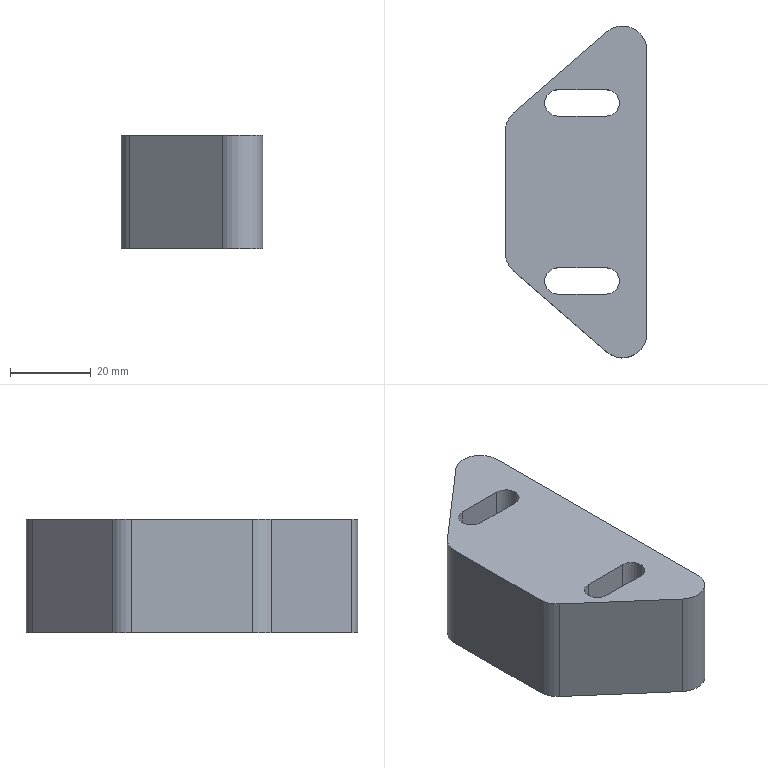Component | SolidWorks | DoubleFilmTransport-1_SynchronousBeltPressureBlock-1 | 1 solid | 19 faces | box 35 x 82 x 28 mm | volume 56182 mm3 | plane 10 | cylinder 9 | commonest cylinder face diameters 12 x5 6.5 x4
build123d program:
from build123d import *

# Parameters (mm, degrees)
BOSS_EXTRUDE1_DEPTH = 28


with BuildPart() as part:
    # Sketch1 → Boss-Extrude1 (new body)
    with BuildSketch(Plane(origin=(0, 0, -14), x_dir=(-1, 0, 0), z_dir=(0, 0, -1))):
        with BuildLine():
            Line((35, 0), (-35, 0))
            ThreePointArc((-35, 0), (-40.46, -3.512), (-39.528, -9.937))
            Line((-39.528, -9.937), (-19.528, -32.937))
            ThreePointArc((-19.528, -32.937), (-17.488, -34.46), (-15, -35))
            Line((-15, -35), (15, -35))
            ThreePointArc((15, -35), (17.488, -34.46), (19.528, -32.937))
            Line((19.528, -32.937), (39.528, -9.937))
            ThreePointArc((39.528, -9.937), (40.46, -3.512), (35, 0))
        make_face()
        with BuildLine():
            Line((18.75, -22), (18.75, -10))
            ThreePointArc((18.75, -10), (22, -6.75), (25.25, -10))
            Line((25.25, -10), (25.25, -22))
            ThreePointArc((25.25, -22), (22, -25.25), (18.75, -22))
        make_face(mode=Mode.SUBTRACT)
        with BuildLine():
            Line((-25.25, -22), (-25.25, -10))
            ThreePointArc((-25.25, -10), (-22, -6.75), (-18.75, -10))
            Line((-18.75, -10), (-18.75, -22))
            ThreePointArc((-18.75, -22), (-22, -25.25), (-25.25, -22))
        make_face(mode=Mode.SUBTRACT)
    extrude(amount=-BOSS_EXTRUDE1_DEPTH)


solid = part.part

# Placed as in the assembly
solid = solid.moved(Location((-356.177, 174.373, 110), (0, 0, -90)))
STEP:
#1=COLOUR_RGB('',0.7922,0.8196,0.9333);
#2=FILL_AREA_STYLE_COLOUR('',#1);
#3=FILL_AREA_STYLE('',(#2));
#4=SURFACE_STYLE_FILL_AREA(#3);
#5=SURFACE_SIDE_STYLE('',(#4));
#6=SURFACE_STYLE_USAGE(.BOTH.,#5);
#7=PRESENTATION_STYLE_ASSIGNMENT((#6));
#8=CARTESIAN_POINT('',(-14.414,8.421,4.882));
#9=VERTEX_POINT('',#8);
#10=CARTESIAN_POINT('',(-14.259,8.479,4.882));
#11=VERTEX_POINT('',#10);
#12=CARTESIAN_POINT('',(-14.259,8.243,4.882));
#13=DIRECTION('',(0.,0.,-1.));
#14=DIRECTION('',(0.,1.,0.));
#15=AXIS2_PLACEMENT_3D('',#12,#13,#14);
#16=CIRCLE('',#15,0.2362);
#17=EDGE_CURVE('',#9,#11,#16,.T.);
#18=ORIENTED_EDGE('',*,*,#17,.T.);
#19=CARTESIAN_POINT('',(-14.259,8.479,3.78));
#20=VERTEX_POINT('',#19);
#21=CARTESIAN_POINT('',(-14.259,8.479,4.882));
#22=DIRECTION('',(0.,0.,-1.));
#23=VECTOR('',#22,39.37);
#24=LINE('',#21,#23);
#25=EDGE_CURVE('',#11,#20,#24,.T.);
#26=ORIENTED_EDGE('',*,*,#25,.T.);
#27=CARTESIAN_POINT('',(-14.414,8.421,3.78));
#28=VERTEX_POINT('',#27);
#29=CARTESIAN_POINT('',(-14.259,8.243,3.78));
#30=DIRECTION('',(0.,0.,-1.));
#31=DIRECTION('',(0.,1.,0.));
#32=AXIS2_PLACEMENT_3D('',#29,#30,#31);
#33=CIRCLE('',#32,0.2362);
#34=EDGE_CURVE('',#28,#20,#33,.T.);
#35=ORIENTED_EDGE('',*,*,#34,.F.);
#36=CARTESIAN_POINT('',(-14.414,8.421,4.882));
#37=DIRECTION('',(0.,0.,-1.));
#38=VECTOR('',#37,39.37);
#39=LINE('',#36,#38);
#40=EDGE_CURVE('',#9,#28,#39,.T.);
#41=ORIENTED_EDGE('',*,*,#40,.F.);
#42=EDGE_LOOP('',(#18,#26,#35,#41));
#43=FACE_OUTER_BOUND('',#42,.T.);
#44=CARTESIAN_POINT('',(-14.259,8.243,4.882));
#45=DIRECTION('',(0.,0.,-1.));
#46=DIRECTION('',(0.,1.,0.));
#47=AXIS2_PLACEMENT_3D('',#44,#45,#46);
#48=CYLINDRICAL_SURFACE('',#47,0.2362);
#49=ADVANCED_FACE('',(#43),#48,.T.);
#50=ORIENTED_EDGE('',*,*,#25,.F.);
#51=CARTESIAN_POINT('',(-14.023,8.243,4.882));
#52=VERTEX_POINT('',#51);
#53=CARTESIAN_POINT('',(-14.259,8.243,4.882));
#54=DIRECTION('',(0.,0.,-1.));
#55=DIRECTION('',(0.,1.,0.));
#56=AXIS2_PLACEMENT_3D('',#53,#54,#55);
#57=CIRCLE('',#56,0.2362);
#58=EDGE_CURVE('',#11,#52,#57,.T.);
#59=ORIENTED_EDGE('',*,*,#58,.T.);
#60=CARTESIAN_POINT('',(-14.023,8.243,3.78));
#61=VERTEX_POINT('',#60);
#62=CARTESIAN_POINT('',(-14.023,8.243,4.882));
#63=DIRECTION('',(0.,0.,-1.));
#64=VECTOR('',#63,39.37);
#65=LINE('',#62,#64);
#66=EDGE_CURVE('',#52,#61,#65,.T.);
#67=ORIENTED_EDGE('',*,*,#66,.T.);
#68=CARTESIAN_POINT('',(-14.259,8.243,3.78));
#69=DIRECTION('',(0.,0.,-1.));
#70=DIRECTION('',(0.,1.,0.));
#71=AXIS2_PLACEMENT_3D('',#68,#69,#70);
#72=CIRCLE('',#71,0.2362);
#73=EDGE_CURVE('',#20,#61,#72,.T.);
#74=ORIENTED_EDGE('',*,*,#73,.F.);
#75=EDGE_LOOP('',(#50,#59,#67,#74));
#76=FACE_OUTER_BOUND('',#75,.T.);
#77=CARTESIAN_POINT('',(-14.259,8.243,4.882));
#78=DIRECTION('',(0.,0.,-1.));
#79=DIRECTION('',(0.,1.,0.));
#80=AXIS2_PLACEMENT_3D('',#77,#78,#79);
#81=CYLINDRICAL_SURFACE('',#80,0.2362);
#82=ADVANCED_FACE('',(#76),#81,.T.);
#83=CARTESIAN_POINT('',(-15.319,7.634,3.78));
#84=VERTEX_POINT('',#83);
#85=CARTESIAN_POINT('',(-15.319,7.634,3.78));
#86=DIRECTION('',(0.7546,0.6562,0.));
#87=VECTOR('',#86,39.37);
#88=LINE('',#85,#87);
#89=EDGE_CURVE('',#84,#28,#88,.T.);
#90=ORIENTED_EDGE('',*,*,#89,.F.);
#91=CARTESIAN_POINT('',(-15.319,7.634,4.882));
#92=VERTEX_POINT('',#91);
#93=CARTESIAN_POINT('',(-15.319,7.634,4.882));
#94=DIRECTION('',(0.,0.,-1.));
#95=VECTOR('',#94,39.37);
#96=LINE('',#93,#95);
#97=EDGE_CURVE('',#92,#84,#96,.T.);
#98=ORIENTED_EDGE('',*,*,#97,.F.);
#99=CARTESIAN_POINT('',(-15.319,7.634,4.882));
#100=DIRECTION('',(0.7546,0.6562,0.));
#101=VECTOR('',#100,39.37);
#102=LINE('',#99,#101);
#103=EDGE_CURVE('',#92,#9,#102,.T.);
#104=ORIENTED_EDGE('',*,*,#103,.T.);
#105=ORIENTED_EDGE('',*,*,#40,.T.);
#106=EDGE_LOOP('',(#90,#98,#104,#105));
#107=FACE_OUTER_BOUND('',#106,.T.);
#108=CARTESIAN_POINT('',(-15.319,7.634,4.882));
#109=DIRECTION('',(-0.6562,0.7546,0.));
#110=DIRECTION('',(-0.7546,-0.6562,0.));
#111=AXIS2_PLACEMENT_3D('',#108,#109,#110);
#112=PLANE('',#111);
#113=ADVANCED_FACE('',(#107),#112,.T.);
#114=CARTESIAN_POINT('',(-15.401,7.456,3.78));
#115=VERTEX_POINT('',#114);
#116=CARTESIAN_POINT('',(-15.164,7.456,3.78));
#117=DIRECTION('',(0.,0.,-1.));
#118=DIRECTION('',(0.,1.,0.));
#119=AXIS2_PLACEMENT_3D('',#116,#117,#118);
#120=CIRCLE('',#119,0.2362);
#121=EDGE_CURVE('',#115,#84,#120,.T.);
#122=ORIENTED_EDGE('',*,*,#121,.F.);
#123=CARTESIAN_POINT('',(-15.401,7.456,4.882));
#124=VERTEX_POINT('',#123);
#125=CARTESIAN_POINT('',(-15.401,7.456,4.882));
#126=DIRECTION('',(0.,0.,-1.));
#127=VECTOR('',#126,39.37);
#128=LINE('',#125,#127);
#129=EDGE_CURVE('',#124,#115,#128,.T.);
#130=ORIENTED_EDGE('',*,*,#129,.F.);
#131=CARTESIAN_POINT('',(-15.164,7.456,4.882));
#132=DIRECTION('',(0.,0.,-1.));
#133=DIRECTION('',(0.,1.,0.));
#134=AXIS2_PLACEMENT_3D('',#131,#132,#133);
#135=CIRCLE('',#134,0.2362);
#136=EDGE_CURVE('',#124,#92,#135,.T.);
#137=ORIENTED_EDGE('',*,*,#136,.T.);
#138=ORIENTED_EDGE('',*,*,#97,.T.);
#139=EDGE_LOOP('',(#122,#130,#137,#138));
#140=FACE_OUTER_BOUND('',#139,.T.);
#141=CARTESIAN_POINT('',(-15.164,7.456,4.882));
#142=DIRECTION('',(0.,0.,-1.));
#143=DIRECTION('',(0.,1.,0.));
#144=AXIS2_PLACEMENT_3D('',#141,#142,#143);
#145=CYLINDRICAL_SURFACE('',#144,0.2362);
#146=ADVANCED_FACE('',(#140),#145,.T.);
#147=CARTESIAN_POINT('',(-15.401,6.275,3.78));
#148=VERTEX_POINT('',#147);
#149=CARTESIAN_POINT('',(-15.401,6.275,3.78));
#150=DIRECTION('',(0.,1.,0.));
#151=VECTOR('',#150,39.37);
#152=LINE('',#149,#151);
#153=EDGE_CURVE('',#148,#115,#152,.T.);
#154=ORIENTED_EDGE('',*,*,#153,.F.);
#155=CARTESIAN_POINT('',(-15.401,6.275,4.882));
#156=VERTEX_POINT('',#155);
#157=CARTESIAN_POINT('',(-15.401,6.275,4.882));
#158=DIRECTION('',(0.,0.,-1.));
#159=VECTOR('',#158,39.37);
#160=LINE('',#157,#159);
#161=EDGE_CURVE('',#156,#148,#160,.T.);
#162=ORIENTED_EDGE('',*,*,#161,.F.);
#163=CARTESIAN_POINT('',(-15.401,6.275,4.882));
#164=DIRECTION('',(0.,1.,0.));
#165=VECTOR('',#164,39.37);
#166=LINE('',#163,#165);
#167=EDGE_CURVE('',#156,#124,#166,.T.);
#168=ORIENTED_EDGE('',*,*,#167,.T.);
#169=ORIENTED_EDGE('',*,*,#129,.T.);
#170=EDGE_LOOP('',(#154,#162,#168,#169));
#171=FACE_OUTER_BOUND('',#170,.T.);
#172=CARTESIAN_POINT('',(-15.401,6.275,4.882));
#173=DIRECTION('',(-1.,0.,0.));
#174=DIRECTION('',(0.,0.,-1.));
#175=AXIS2_PLACEMENT_3D('',#172,#173,#174);
#176=PLANE('',#175);
#177=ADVANCED_FACE('',(#171),#176,.T.);
#178=CARTESIAN_POINT('',(-15.319,6.096,3.78));
#179=VERTEX_POINT('',#178);
#180=CARTESIAN_POINT('',(-15.164,6.275,3.78));
#181=DIRECTION('',(0.,0.,-1.));
#182=DIRECTION('',(0.,1.,0.));
#183=AXIS2_PLACEMENT_3D('',#180,#181,#182);
#184=CIRCLE('',#183,0.2362);
#185=EDGE_CURVE('',#179,#148,#184,.T.);
#186=ORIENTED_EDGE('',*,*,#185,.F.);
#187=CARTESIAN_POINT('',(-15.319,6.096,4.882));
#188=VERTEX_POINT('',#187);
#189=CARTESIAN_POINT('',(-15.319,6.096,4.882));
#190=DIRECTION('',(0.,0.,-1.));
#191=VECTOR('',#190,39.37);
#192=LINE('',#189,#191);
#193=EDGE_CURVE('',#188,#179,#192,.T.);
#194=ORIENTED_EDGE('',*,*,#193,.F.);
#195=CARTESIAN_POINT('',(-15.164,6.275,4.882));
#196=DIRECTION('',(0.,0.,-1.));
#197=DIRECTION('',(0.,1.,0.));
#198=AXIS2_PLACEMENT_3D('',#195,#196,#197);
#199=CIRCLE('',#198,0.2362);
#200=EDGE_CURVE('',#188,#156,#199,.T.);
#201=ORIENTED_EDGE('',*,*,#200,.T.);
#202=ORIENTED_EDGE('',*,*,#161,.T.);
#203=EDGE_LOOP('',(#186,#194,#201,#202));
#204=FACE_OUTER_BOUND('',#203,.T.);
#205=CARTESIAN_POINT('',(-15.164,6.275,4.882));
#206=DIRECTION('',(0.,0.,-1.));
#207=DIRECTION('',(0.,1.,0.));
#208=AXIS2_PLACEMENT_3D('',#205,#206,#207);
#209=CYLINDRICAL_SURFACE('',#208,0.2362);
#210=ADVANCED_FACE('',(#204),#209,.T.);
#211=CARTESIAN_POINT('',(-14.414,5.309,3.78));
#212=VERTEX_POINT('',#211);
#213=CARTESIAN_POINT('',(-14.414,5.309,3.78));
#214=DIRECTION('',(-0.7546,0.6562,0.));
#215=VECTOR('',#214,39.37);
#216=LINE('',#213,#215);
#217=EDGE_CURVE('',#212,#179,#216,.T.);
#218=ORIENTED_EDGE('',*,*,#217,.F.);
#219=CARTESIAN_POINT('',(-14.414,5.309,4.882));
#220=VERTEX_POINT('',#219);
#221=CARTESIAN_POINT('',(-14.414,5.309,4.882));
#222=DIRECTION('',(0.,0.,-1.));
#223=VECTOR('',#222,39.37);
#224=LINE('',#221,#223);
#225=EDGE_CURVE('',#220,#212,#224,.T.);
#226=ORIENTED_EDGE('',*,*,#225,.F.);
#227=CARTESIAN_POINT('',(-14.414,5.309,4.882));
#228=DIRECTION('',(-0.7546,0.6562,0.));
#229=VECTOR('',#228,39.37);
#230=LINE('',#227,#229);
#231=EDGE_CURVE('',#220,#188,#230,.T.);
#232=ORIENTED_EDGE('',*,*,#231,.T.);
#233=ORIENTED_EDGE('',*,*,#193,.T.);
#234=EDGE_LOOP('',(#218,#226,#232,#233));
#235=FACE_OUTER_BOUND('',#234,.T.);
#236=CARTESIAN_POINT('',(-14.414,5.309,4.882));
#237=DIRECTION('',(-0.6562,-0.7546,0.));
#238=DIRECTION('',(0.7546,-0.6562,0.));
#239=AXIS2_PLACEMENT_3D('',#236,#237,#238);
#240=PLANE('',#239);
#241=ADVANCED_FACE('',(#235),#240,.T.);
#242=CARTESIAN_POINT('',(-14.023,5.487,3.78));
#243=VERTEX_POINT('',#242);
#244=CARTESIAN_POINT('',(-14.259,5.487,3.78));
#245=DIRECTION('',(0.,0.,-1.));
#246=DIRECTION('',(0.,1.,0.));
#247=AXIS2_PLACEMENT_3D('',#244,#245,#246);
#248=CIRCLE('',#247,0.2362);
#249=EDGE_CURVE('',#243,#212,#248,.T.);
#250=ORIENTED_EDGE('',*,*,#249,.F.);
#251=CARTESIAN_POINT('',(-14.023,5.487,4.882));
#252=VERTEX_POINT('',#251);
#253=CARTESIAN_POINT('',(-14.023,5.487,4.882));
#254=DIRECTION('',(0.,0.,-1.));
#255=VECTOR('',#254,39.37);
#256=LINE('',#253,#255);
#257=EDGE_CURVE('',#252,#243,#256,.T.);
#258=ORIENTED_EDGE('',*,*,#257,.F.);
#259=CARTESIAN_POINT('',(-14.259,5.487,4.882));
#260=DIRECTION('',(0.,0.,-1.));
#261=DIRECTION('',(0.,1.,0.));
#262=AXIS2_PLACEMENT_3D('',#259,#260,#261);
#263=CIRCLE('',#262,0.2362);
#264=EDGE_CURVE('',#252,#220,#263,.T.);
#265=ORIENTED_EDGE('',*,*,#264,.T.);
#266=ORIENTED_EDGE('',*,*,#225,.T.);
#267=EDGE_LOOP('',(#250,#258,#265,#266));
#268=FACE_OUTER_BOUND('',#267,.T.);
#269=CARTESIAN_POINT('',(-14.259,5.487,4.882));
#270=DIRECTION('',(0.,0.,-1.));
#271=DIRECTION('',(0.,1.,0.));
#272=AXIS2_PLACEMENT_3D('',#269,#270,#271);
#273=CYLINDRICAL_SURFACE('',#272,0.2362);
#274=ADVANCED_FACE('',(#268),#273,.T.);
#275=CARTESIAN_POINT('',(-14.023,8.243,3.78));
#276=DIRECTION('',(-0.,-1.,0.));
#277=VECTOR('',#276,39.37);
#278=LINE('',#275,#277);
#279=EDGE_CURVE('',#61,#243,#278,.T.);
#280=ORIENTED_EDGE('',*,*,#279,.F.);
#281=ORIENTED_EDGE('',*,*,#66,.F.);
#282=CARTESIAN_POINT('',(-14.023,8.243,4.882));
#283=DIRECTION('',(-0.,-1.,0.));
#284=VECTOR('',#283,39.37);
#285=LINE('',#282,#284);
#286=EDGE_CURVE('',#52,#252,#285,.T.);
#287=ORIENTED_EDGE('',*,*,#286,.T.);
#288=ORIENTED_EDGE('',*,*,#257,.T.);
#289=EDGE_LOOP('',(#280,#281,#287,#288));
#290=FACE_OUTER_BOUND('',#289,.T.);
#291=CARTESIAN_POINT('',(-14.023,8.243,4.882));
#292=DIRECTION('',(1.,-0.,0.));
#293=DIRECTION('',(0.,1.,0.));
#294=AXIS2_PLACEMENT_3D('',#291,#292,#293);
#295=PLANE('',#294);
#296=ADVANCED_FACE('',(#290),#295,.T.);
#297=CARTESIAN_POINT('',(-14.416,5.871,4.882));
#298=VERTEX_POINT('',#297);
#299=CARTESIAN_POINT('',(-14.889,5.871,4.882));
#300=VERTEX_POINT('',#299);
#301=CARTESIAN_POINT('',(-14.889,5.871,4.882));
#302=DIRECTION('',(-1.,0.,0.));
#303=VECTOR('',#302,39.37);
#304=LINE('',#301,#303);
#305=EDGE_CURVE('',#298,#300,#304,.T.);
#306=ORIENTED_EDGE('',*,*,#305,.T.);
#307=CARTESIAN_POINT('',(-14.889,6.127,4.882));
#308=VERTEX_POINT('',#307);
#309=CARTESIAN_POINT('',(-14.889,5.999,4.882));
#310=DIRECTION('',(0.,0.,-1.));
#311=DIRECTION('',(0.,-1.,0.));
#312=AXIS2_PLACEMENT_3D('',#309,#310,#311);
#313=CIRCLE('',#312,0.128);
#314=EDGE_CURVE('',#300,#308,#313,.T.);
#315=ORIENTED_EDGE('',*,*,#314,.T.);
#316=CARTESIAN_POINT('',(-14.416,6.127,4.882));
#317=VERTEX_POINT('',#316);
#318=CARTESIAN_POINT('',(-14.416,6.127,4.882));
#319=DIRECTION('',(1.,-0.,0.));
#320=VECTOR('',#319,39.37);
#321=LINE('',#318,#320);
#322=EDGE_CURVE('',#308,#317,#321,.T.);
#323=ORIENTED_EDGE('',*,*,#322,.T.);
#324=CARTESIAN_POINT('',(-14.416,5.999,4.882));
#325=DIRECTION('',(0.,0.,-1.));
#326=DIRECTION('',(0.,-1.,0.));
#327=AXIS2_PLACEMENT_3D('',#324,#325,#326);
#328=CIRCLE('',#327,0.128);
#329=EDGE_CURVE('',#317,#298,#328,.T.);
#330=ORIENTED_EDGE('',*,*,#329,.T.);
#331=EDGE_LOOP('',(#306,#315,#323,#330));
#332=FACE_BOUND('',#331,.T.);
#333=CARTESIAN_POINT('',(-14.416,7.603,4.882));
#334=VERTEX_POINT('',#333);
#335=CARTESIAN_POINT('',(-14.889,7.603,4.882));
#336=VERTEX_POINT('',#335);
#337=CARTESIAN_POINT('',(-14.889,7.603,4.882));
#338=DIRECTION('',(-1.,0.,0.));
#339=VECTOR('',#338,39.37);
#340=LINE('',#337,#339);
#341=EDGE_CURVE('',#334,#336,#340,.T.);
#342=ORIENTED_EDGE('',*,*,#341,.T.);
#343=CARTESIAN_POINT('',(-14.889,7.859,4.882));
#344=VERTEX_POINT('',#343);
#345=CARTESIAN_POINT('',(-14.889,7.731,4.882));
#346=DIRECTION('',(0.,0.,-1.));
#347=DIRECTION('',(0.,-1.,0.));
#348=AXIS2_PLACEMENT_3D('',#345,#346,#347);
#349=CIRCLE('',#348,0.128);
#350=EDGE_CURVE('',#336,#344,#349,.T.);
#351=ORIENTED_EDGE('',*,*,#350,.T.);
#352=CARTESIAN_POINT('',(-14.416,7.859,4.882));
#353=VERTEX_POINT('',#352);
#354=CARTESIAN_POINT('',(-14.416,7.859,4.882));
#355=DIRECTION('',(1.,-0.,0.));
#356=VECTOR('',#355,39.37);
#357=LINE('',#354,#356);
#358=EDGE_CURVE('',#344,#353,#357,.T.);
#359=ORIENTED_EDGE('',*,*,#358,.T.);
#360=CARTESIAN_POINT('',(-14.416,7.731,4.882));
#361=DIRECTION('',(0.,0.,-1.));
#362=DIRECTION('',(0.,-1.,0.));
#363=AXIS2_PLACEMENT_3D('',#360,#361,#362);
#364=CIRCLE('',#363,0.128);
#365=EDGE_CURVE('',#353,#334,#364,.T.);
#366=ORIENTED_EDGE('',*,*,#365,.T.);
#367=EDGE_LOOP('',(#342,#351,#359,#366));
#368=FACE_BOUND('',#367,.T.);
#369=ORIENTED_EDGE('',*,*,#17,.F.);
#370=ORIENTED_EDGE('',*,*,#103,.F.);
#371=ORIENTED_EDGE('',*,*,#136,.F.);
#372=ORIENTED_EDGE('',*,*,#167,.F.);
#373=ORIENTED_EDGE('',*,*,#200,.F.);
#374=ORIENTED_EDGE('',*,*,#231,.F.);
#375=ORIENTED_EDGE('',*,*,#264,.F.);
#376=ORIENTED_EDGE('',*,*,#286,.F.);
#377=ORIENTED_EDGE('',*,*,#58,.F.);
#378=EDGE_LOOP('',(#369,#370,#371,#372,#373,#374,#375,#376,#377));
#379=FACE_OUTER_BOUND('',#378,.T.);
#380=CARTESIAN_POINT('',(-14.259,8.243,4.882));
#381=DIRECTION('',(0.,0.,-1.));
#382=DIRECTION('',(0.,1.,0.));
#383=AXIS2_PLACEMENT_3D('',#380,#381,#382);
#384=PLANE('',#383);
#385=ADVANCED_FACE('',(#332,#368,#379),#384,.F.);
#386=CARTESIAN_POINT('',(-14.889,5.871,3.78));
#387=VERTEX_POINT('',#386);
#388=CARTESIAN_POINT('',(-14.889,6.127,3.78));
#389=VERTEX_POINT('',#388);
#390=CARTESIAN_POINT('',(-14.889,5.999,3.78));
#391=DIRECTION('',(0.,0.,-1.));
#392=DIRECTION('',(0.,-1.,0.));
#393=AXIS2_PLACEMENT_3D('',#390,#391,#392);
#394=CIRCLE('',#393,0.128);
#395=EDGE_CURVE('',#387,#389,#394,.T.);
#396=ORIENTED_EDGE('',*,*,#395,.F.);
#397=CARTESIAN_POINT('',(-14.416,5.871,3.78));
#398=VERTEX_POINT('',#397);
#399=CARTESIAN_POINT('',(-14.889,5.871,3.78));
#400=DIRECTION('',(-1.,0.,0.));
#401=VECTOR('',#400,39.37);
#402=LINE('',#399,#401);
#403=EDGE_CURVE('',#398,#387,#402,.T.);
#404=ORIENTED_EDGE('',*,*,#403,.F.);
#405=CARTESIAN_POINT('',(-14.416,6.127,3.78));
#406=VERTEX_POINT('',#405);
#407=CARTESIAN_POINT('',(-14.416,5.999,3.78));
#408=DIRECTION('',(0.,0.,-1.));
#409=DIRECTION('',(0.,-1.,0.));
#410=AXIS2_PLACEMENT_3D('',#407,#408,#409);
#411=CIRCLE('',#410,0.128);
#412=EDGE_CURVE('',#406,#398,#411,.T.);
#413=ORIENTED_EDGE('',*,*,#412,.F.);
#414=CARTESIAN_POINT('',(-14.416,6.127,3.78));
#415=DIRECTION('',(1.,-0.,0.));
#416=VECTOR('',#415,39.37);
#417=LINE('',#414,#416);
#418=EDGE_CURVE('',#389,#406,#417,.T.);
#419=ORIENTED_EDGE('',*,*,#418,.F.);
#420=EDGE_LOOP('',(#396,#404,#413,#419));
#421=FACE_BOUND('',#420,.T.);
#422=CARTESIAN_POINT('',(-14.889,7.603,3.78));
#423=VERTEX_POINT('',#422);
#424=CARTESIAN_POINT('',(-14.889,7.859,3.78));
#425=VERTEX_POINT('',#424);
#426=CARTESIAN_POINT('',(-14.889,7.731,3.78));
#427=DIRECTION('',(0.,0.,-1.));
#428=DIRECTION('',(0.,-1.,0.));
#429=AXIS2_PLACEMENT_3D('',#426,#427,#428);
#430=CIRCLE('',#429,0.128);
#431=EDGE_CURVE('',#423,#425,#430,.T.);
#432=ORIENTED_EDGE('',*,*,#431,.F.);
#433=CARTESIAN_POINT('',(-14.416,7.603,3.78));
#434=VERTEX_POINT('',#433);
#435=CARTESIAN_POINT('',(-14.889,7.603,3.78));
#436=DIRECTION('',(-1.,0.,0.));
#437=VECTOR('',#436,39.37);
#438=LINE('',#435,#437);
#439=EDGE_CURVE('',#434,#423,#438,.T.);
#440=ORIENTED_EDGE('',*,*,#439,.F.);
#441=CARTESIAN_POINT('',(-14.416,7.859,3.78));
#442=VERTEX_POINT('',#441);
#443=CARTESIAN_POINT('',(-14.416,7.731,3.78));
#444=DIRECTION('',(0.,0.,-1.));
#445=DIRECTION('',(0.,-1.,0.));
#446=AXIS2_PLACEMENT_3D('',#443,#444,#445);
#447=CIRCLE('',#446,0.128);
#448=EDGE_CURVE('',#442,#434,#447,.T.);
#449=ORIENTED_EDGE('',*,*,#448,.F.);
#450=CARTESIAN_POINT('',(-14.416,7.859,3.78));
#451=DIRECTION('',(1.,-0.,0.));
#452=VECTOR('',#451,39.37);
#453=LINE('',#450,#452);
#454=EDGE_CURVE('',#425,#442,#453,.T.);
#455=ORIENTED_EDGE('',*,*,#454,.F.);
#456=EDGE_LOOP('',(#432,#440,#449,#455));
#457=FACE_BOUND('',#456,.T.);
#458=ORIENTED_EDGE('',*,*,#34,.T.);
#459=ORIENTED_EDGE('',*,*,#73,.T.);
#460=ORIENTED_EDGE('',*,*,#279,.T.);
#461=ORIENTED_EDGE('',*,*,#249,.T.);
#462=ORIENTED_EDGE('',*,*,#217,.T.);
#463=ORIENTED_EDGE('',*,*,#185,.T.);
#464=ORIENTED_EDGE('',*,*,#153,.T.);
#465=ORIENTED_EDGE('',*,*,#121,.T.);
#466=ORIENTED_EDGE('',*,*,#89,.T.);
#467=EDGE_LOOP('',(#458,#459,#460,#461,#462,#463,#464,#465,#466));
#468=FACE_OUTER_BOUND('',#467,.T.);
#469=CARTESIAN_POINT('',(-14.259,8.243,3.78));
#470=DIRECTION('',(0.,0.,-1.));
#471=DIRECTION('',(0.,1.,0.));
#472=AXIS2_PLACEMENT_3D('',#469,#470,#471);
#473=PLANE('',#472);
#474=ADVANCED_FACE('',(#421,#457,#468),#473,.T.);
#475=ORIENTED_EDGE('',*,*,#431,.T.);
#476=CARTESIAN_POINT('',(-14.889,7.859,4.882));
#477=DIRECTION('',(0.,0.,-1.));
#478=VECTOR('',#477,39.37);
#479=LINE('',#476,#478);
#480=EDGE_CURVE('',#344,#425,#479,.T.);
#481=ORIENTED_EDGE('',*,*,#480,.F.);
#482=ORIENTED_EDGE('',*,*,#350,.F.);
#483=CARTESIAN_POINT('',(-14.889,7.603,4.882));
#484=DIRECTION('',(0.,0.,-1.));
#485=VECTOR('',#484,39.37);
#486=LINE('',#483,#485);
#487=EDGE_CURVE('',#336,#423,#486,.T.);
#488=ORIENTED_EDGE('',*,*,#487,.T.);
#489=EDGE_LOOP('',(#475,#481,#482,#488));
#490=FACE_OUTER_BOUND('',#489,.T.);
#491=CARTESIAN_POINT('',(-14.889,7.731,4.882));
#492=DIRECTION('',(0.,0.,-1.));
#493=DIRECTION('',(0.,1.,0.));
#494=AXIS2_PLACEMENT_3D('',#491,#492,#493);
#495=CYLINDRICAL_SURFACE('',#494,0.128);
#496=ADVANCED_FACE('',(#490),#495,.F.);
#497=ORIENTED_EDGE('',*,*,#439,.T.);
#498=ORIENTED_EDGE('',*,*,#487,.F.);
#499=ORIENTED_EDGE('',*,*,#341,.F.);
#500=CARTESIAN_POINT('',(-14.416,7.603,4.882));
#501=DIRECTION('',(0.,0.,-1.));
#502=VECTOR('',#501,39.37);
#503=LINE('',#500,#502);
#504=EDGE_CURVE('',#334,#434,#503,.T.);
#505=ORIENTED_EDGE('',*,*,#504,.T.);
#506=EDGE_LOOP('',(#497,#498,#499,#505));
#507=FACE_OUTER_BOUND('',#506,.T.);
#508=CARTESIAN_POINT('',(-14.889,7.603,4.882));
#509=DIRECTION('',(-0.,-1.,0.));
#510=DIRECTION('',(0.,0.,-1.));
#511=AXIS2_PLACEMENT_3D('',#508,#509,#510);
#512=PLANE('',#511);
#513=ADVANCED_FACE('',(#507),#512,.F.);
#514=ORIENTED_EDGE('',*,*,#448,.T.);
#515=ORIENTED_EDGE('',*,*,#504,.F.);
#516=ORIENTED_EDGE('',*,*,#365,.F.);
#517=CARTESIAN_POINT('',(-14.416,7.859,4.882));
#518=DIRECTION('',(0.,0.,-1.));
#519=VECTOR('',#518,39.37);
#520=LINE('',#517,#519);
#521=EDGE_CURVE('',#353,#442,#520,.T.);
#522=ORIENTED_EDGE('',*,*,#521,.T.);
#523=EDGE_LOOP('',(#514,#515,#516,#522));
#524=FACE_OUTER_BOUND('',#523,.T.);
#525=CARTESIAN_POINT('',(-14.416,7.731,4.882));
#526=DIRECTION('',(0.,0.,-1.));
#527=DIRECTION('',(0.,1.,0.));
#528=AXIS2_PLACEMENT_3D('',#525,#526,#527);
#529=CYLINDRICAL_SURFACE('',#528,0.128);
#530=ADVANCED_FACE('',(#524),#529,.F.);
#531=ORIENTED_EDGE('',*,*,#454,.T.);
#532=ORIENTED_EDGE('',*,*,#521,.F.);
#533=ORIENTED_EDGE('',*,*,#358,.F.);
#534=ORIENTED_EDGE('',*,*,#480,.T.);
#535=EDGE_LOOP('',(#531,#532,#533,#534));
#536=FACE_OUTER_BOUND('',#535,.T.);
#537=CARTESIAN_POINT('',(-14.416,7.859,4.882));
#538=DIRECTION('',(0.,1.,0.));
#539=DIRECTION('',(0.,0.,1.));
#540=AXIS2_PLACEMENT_3D('',#537,#538,#539);
#541=PLANE('',#540);
#542=ADVANCED_FACE('',(#536),#541,.F.);
#543=ORIENTED_EDGE('',*,*,#395,.T.);
#544=CARTESIAN_POINT('',(-14.889,6.127,4.882));
#545=DIRECTION('',(0.,0.,-1.));
#546=VECTOR('',#545,39.37);
#547=LINE('',#544,#546);
#548=EDGE_CURVE('',#308,#389,#547,.T.);
#549=ORIENTED_EDGE('',*,*,#548,.F.);
#550=ORIENTED_EDGE('',*,*,#314,.F.);
#551=CARTESIAN_POINT('',(-14.889,5.871,4.882));
#552=DIRECTION('',(0.,0.,-1.));
#553=VECTOR('',#552,39.37);
#554=LINE('',#551,#553);
#555=EDGE_CURVE('',#300,#387,#554,.T.);
#556=ORIENTED_EDGE('',*,*,#555,.T.);
#557=EDGE_LOOP('',(#543,#549,#550,#556));
#558=FACE_OUTER_BOUND('',#557,.T.);
#559=CARTESIAN_POINT('',(-14.889,5.999,4.882));
#560=DIRECTION('',(0.,0.,-1.));
#561=DIRECTION('',(0.,1.,0.));
#562=AXIS2_PLACEMENT_3D('',#559,#560,#561);
#563=CYLINDRICAL_SURFACE('',#562,0.128);
#564=ADVANCED_FACE('',(#558),#563,.F.);
#565=ORIENTED_EDGE('',*,*,#403,.T.);
#566=ORIENTED_EDGE('',*,*,#555,.F.);
#567=ORIENTED_EDGE('',*,*,#305,.F.);
#568=CARTESIAN_POINT('',(-14.416,5.871,4.882));
#569=DIRECTION('',(0.,0.,-1.));
#570=VECTOR('',#569,39.37);
#571=LINE('',#568,#570);
#572=EDGE_CURVE('',#298,#398,#571,.T.);
#573=ORIENTED_EDGE('',*,*,#572,.T.);
#574=EDGE_LOOP('',(#565,#566,#567,#573));
#575=FACE_OUTER_BOUND('',#574,.T.);
#576=CARTESIAN_POINT('',(-14.889,5.871,4.882));
#577=DIRECTION('',(-0.,-1.,0.));
#578=DIRECTION('',(0.,0.,-1.));
#579=AXIS2_PLACEMENT_3D('',#576,#577,#578);
#580=PLANE('',#579);
#581=ADVANCED_FACE('',(#575),#580,.F.);
#582=ORIENTED_EDGE('',*,*,#412,.T.);
#583=ORIENTED_EDGE('',*,*,#572,.F.);
#584=ORIENTED_EDGE('',*,*,#329,.F.);
#585=CARTESIAN_POINT('',(-14.416,6.127,4.882));
#586=DIRECTION('',(0.,0.,-1.));
#587=VECTOR('',#586,39.37);
#588=LINE('',#585,#587);
#589=EDGE_CURVE('',#317,#406,#588,.T.);
#590=ORIENTED_EDGE('',*,*,#589,.T.);
#591=EDGE_LOOP('',(#582,#583,#584,#590));
#592=FACE_OUTER_BOUND('',#591,.T.);
#593=CARTESIAN_POINT('',(-14.416,5.999,4.882));
#594=DIRECTION('',(0.,0.,-1.));
#595=DIRECTION('',(0.,1.,0.));
#596=AXIS2_PLACEMENT_3D('',#593,#594,#595);
#597=CYLINDRICAL_SURFACE('',#596,0.128);
#598=ADVANCED_FACE('',(#592),#597,.F.);
#599=ORIENTED_EDGE('',*,*,#418,.T.);
#600=ORIENTED_EDGE('',*,*,#589,.F.);
#601=ORIENTED_EDGE('',*,*,#322,.F.);
#602=ORIENTED_EDGE('',*,*,#548,.T.);
#603=EDGE_LOOP('',(#599,#600,#601,#602));
#604=FACE_OUTER_BOUND('',#603,.T.);
#605=CARTESIAN_POINT('',(-14.416,6.127,4.882));
#606=DIRECTION('',(0.,1.,0.));
#607=DIRECTION('',(0.,0.,1.));
#608=AXIS2_PLACEMENT_3D('',#605,#606,#607);
#609=PLANE('',#608);
#610=ADVANCED_FACE('',(#604),#609,.F.);
#611=CLOSED_SHELL('',(#49,#82,#113,#146,#177,#210,#241,#274,#296,#385,#474,#496,#513,#530,#542,#564,#581,#598,#610));
#612=MANIFOLD_SOLID_BREP('',#611);
#613=STYLED_ITEM('',(#7),#612);
#614=(LENGTH_UNIT()NAMED_UNIT(*)SI_UNIT($,.METRE.));
#615=LENGTH_MEASURE_WITH_UNIT(LENGTH_MEASURE(0.0254),#614);
#616=DIMENSIONAL_EXPONENTS(1.,0.,0.,0.,0.,0.,0.);
#617=(CONVERSION_BASED_UNIT('',#615)LENGTH_UNIT()NAMED_UNIT(#616));
#618=UNCERTAINTY_MEASURE_WITH_UNIT(LENGTH_MEASURE(0.00001),#617,'','');
#619=(NAMED_UNIT(*)PLANE_ANGLE_UNIT()SI_UNIT($,.RADIAN.));
#620=(NAMED_UNIT(*)SI_UNIT($,.STERADIAN.)SOLID_ANGLE_UNIT());
#621=(GEOMETRIC_REPRESENTATION_CONTEXT(3)GLOBAL_UNCERTAINTY_ASSIGNED_CONTEXT((#618))GLOBAL_UNIT_ASSIGNED_CONTEXT((#617,#619,#620))REPRESENTATION_CONTEXT('',''));
#622=MECHANICAL_DESIGN_GEOMETRIC_PRESENTATION_REPRESENTATION('',(#613),#621);
#623=CARTESIAN_POINT('',(0.,0.,0.));
#624=DIRECTION('',(0.,0.,1.));
#625=DIRECTION('',(1.,0.,0.));
#626=AXIS2_PLACEMENT_3D('',#623,#624,#625);
#627=(LENGTH_UNIT()NAMED_UNIT(*)SI_UNIT($,.METRE.));
#628=LENGTH_MEASURE_WITH_UNIT(LENGTH_MEASURE(0.0254),#627);
#629=DIMENSIONAL_EXPONENTS(1.,0.,0.,0.,0.,0.,0.);
#630=(CONVERSION_BASED_UNIT('',#628)LENGTH_UNIT()NAMED_UNIT(#629));
#631=UNCERTAINTY_MEASURE_WITH_UNIT(LENGTH_MEASURE(0.00001),#630,'','');
#632=(NAMED_UNIT(*)PLANE_ANGLE_UNIT()SI_UNIT($,.RADIAN.));
#633=(NAMED_UNIT(*)SI_UNIT($,.STERADIAN.)SOLID_ANGLE_UNIT());
#634=(GEOMETRIC_REPRESENTATION_CONTEXT(3)GLOBAL_UNCERTAINTY_ASSIGNED_CONTEXT((#631))GLOBAL_UNIT_ASSIGNED_CONTEXT((#630,#632,#633))REPRESENTATION_CONTEXT('',''));
#635=ADVANCED_BREP_SHAPE_REPRESENTATION('',(#612,#626),#634);
#636=PRESENTATION_LAYER_ASSIGNMENT('','',(#613));